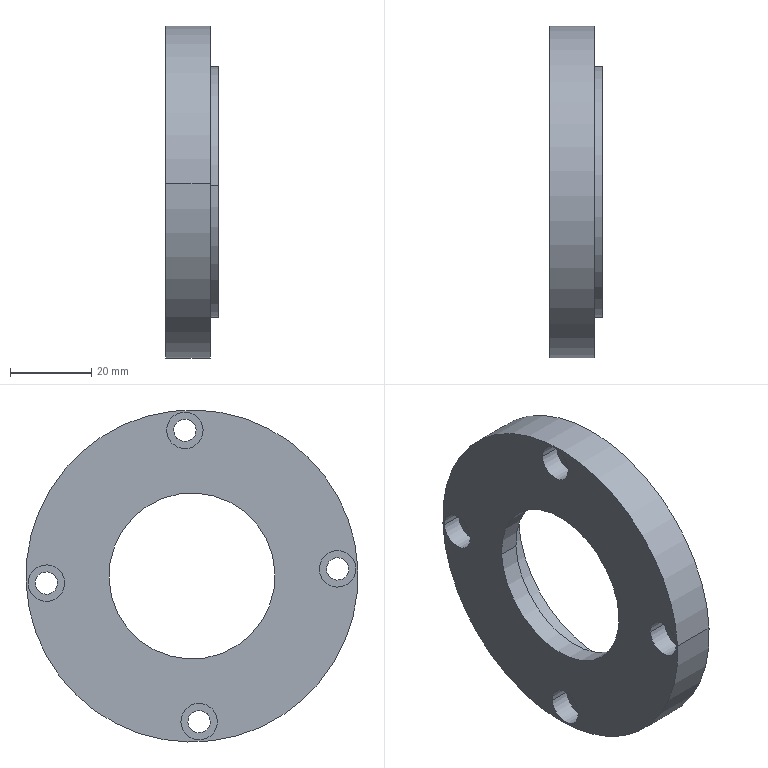Component | SolidWorks | 2-10-10WorkpieceAxisAssembly-1_2-10-3BearingSideCover-2 | 1 solid | 32 faces | box 13 x 82 x 82 mm | volume 36679 mm3 | cylinder 24 | plane 8 | commonest cylinder face diameters 5.5 x8 9 x8 41 x2 55 x2 62 x2 82 x2
STEP:
#1=COLOUR_RGB('',0.7922,0.8196,0.9333);
#2=FILL_AREA_STYLE_COLOUR('',#1);
#3=FILL_AREA_STYLE('',(#2));
#4=SURFACE_STYLE_FILL_AREA(#3);
#5=SURFACE_SIDE_STYLE('',(#4));
#6=SURFACE_STYLE_USAGE(.BOTH.,#5);
#7=PRESENTATION_STYLE_ASSIGNMENT((#6));
#8=CARTESIAN_POINT('',(-18.811,-0.2038,1.421));
#9=VERTEX_POINT('',#8);
#10=CARTESIAN_POINT('',(-18.811,0.01251,1.41));
#11=VERTEX_POINT('',#10);
#12=CARTESIAN_POINT('',(-18.811,-0.09563,1.416));
#13=DIRECTION('',(1.,-0.,0.));
#14=DIRECTION('',(0.,0.9988,-0.04867));
#15=AXIS2_PLACEMENT_3D('',#12,#13,#14);
#16=CIRCLE('',#15,0.1083);
#17=EDGE_CURVE('',#9,#11,#16,.T.);
#18=ORIENTED_EDGE('',*,*,#17,.T.);
#19=CARTESIAN_POINT('',(-19.048,0.01251,1.41));
#20=VERTEX_POINT('',#19);
#21=CARTESIAN_POINT('',(-19.244,0.01251,1.41));
#22=DIRECTION('',(-1.,0.,-0.));
#23=VECTOR('',#22,39.37);
#24=LINE('',#21,#23);
#25=EDGE_CURVE('',#11,#20,#24,.T.);
#26=ORIENTED_EDGE('',*,*,#25,.T.);
#27=CARTESIAN_POINT('',(-19.048,-0.2038,1.421));
#28=VERTEX_POINT('',#27);
#29=CARTESIAN_POINT('',(-19.048,-0.09563,1.416));
#30=DIRECTION('',(-1.,0.,-0.));
#31=DIRECTION('',(0.,-0.9988,0.04867));
#32=AXIS2_PLACEMENT_3D('',#29,#30,#31);
#33=CIRCLE('',#32,0.1083);
#34=EDGE_CURVE('',#20,#28,#33,.T.);
#35=ORIENTED_EDGE('',*,*,#34,.T.);
#36=CARTESIAN_POINT('',(-19.244,-0.2038,1.421));
#37=DIRECTION('',(-1.,0.,-0.));
#38=VECTOR('',#37,39.37);
#39=LINE('',#36,#38);
#40=EDGE_CURVE('',#9,#28,#39,.T.);
#41=ORIENTED_EDGE('',*,*,#40,.F.);
#42=EDGE_LOOP('',(#18,#26,#35,#41));
#43=FACE_OUTER_BOUND('',#42,.T.);
#44=CARTESIAN_POINT('',(-19.244,-0.09563,1.416));
#45=DIRECTION('',(-1.,0.,-0.));
#46=DIRECTION('',(0.,-0.9988,0.04867));
#47=AXIS2_PLACEMENT_3D('',#44,#45,#46);
#48=CYLINDRICAL_SURFACE('',#47,0.1083);
#49=ADVANCED_FACE('',(#43),#48,.F.);
#50=CARTESIAN_POINT('',(-19.048,0.08133,1.407));
#51=VERTEX_POINT('',#50);
#52=CARTESIAN_POINT('',(-19.048,-0.2726,1.424));
#53=VERTEX_POINT('',#52);
#54=CARTESIAN_POINT('',(-19.048,-0.09563,1.416));
#55=DIRECTION('',(-1.,0.,-0.));
#56=DIRECTION('',(0.,-0.9988,0.04867));
#57=AXIS2_PLACEMENT_3D('',#54,#55,#56);
#58=CIRCLE('',#57,0.1772);
#59=EDGE_CURVE('',#51,#53,#58,.T.);
#60=ORIENTED_EDGE('',*,*,#59,.F.);
#61=CARTESIAN_POINT('',(-19.244,0.08133,1.407));
#62=VERTEX_POINT('',#61);
#63=CARTESIAN_POINT('',(-19.244,0.08133,1.407));
#64=DIRECTION('',(-1.,0.,-0.));
#65=VECTOR('',#64,39.37);
#66=LINE('',#63,#65);
#67=EDGE_CURVE('',#51,#62,#66,.T.);
#68=ORIENTED_EDGE('',*,*,#67,.T.);
#69=CARTESIAN_POINT('',(-19.244,-0.2726,1.424));
#70=VERTEX_POINT('',#69);
#71=CARTESIAN_POINT('',(-19.244,-0.09563,1.416));
#72=DIRECTION('',(-1.,0.,-0.));
#73=DIRECTION('',(0.,-0.9988,0.04867));
#74=AXIS2_PLACEMENT_3D('',#71,#72,#73);
#75=CIRCLE('',#74,0.1772);
#76=EDGE_CURVE('',#62,#70,#75,.T.);
#77=ORIENTED_EDGE('',*,*,#76,.T.);
#78=CARTESIAN_POINT('',(-19.244,-0.2726,1.424));
#79=DIRECTION('',(-1.,0.,-0.));
#80=VECTOR('',#79,39.37);
#81=LINE('',#78,#80);
#82=EDGE_CURVE('',#53,#70,#81,.T.);
#83=ORIENTED_EDGE('',*,*,#82,.F.);
#84=EDGE_LOOP('',(#60,#68,#77,#83));
#85=FACE_OUTER_BOUND('',#84,.T.);
#86=CARTESIAN_POINT('',(-19.244,-0.09563,1.416));
#87=DIRECTION('',(-1.,0.,-0.));
#88=DIRECTION('',(0.,-0.9988,0.04867));
#89=AXIS2_PLACEMENT_3D('',#86,#87,#88);
#90=CYLINDRICAL_SURFACE('',#89,0.1772);
#91=ADVANCED_FACE('',(#85),#90,.F.);
#92=CARTESIAN_POINT('',(-18.811,-1.688,0.07425));
#93=VERTEX_POINT('',#92);
#94=CARTESIAN_POINT('',(-18.811,-1.472,0.06371));
#95=VERTEX_POINT('',#94);
#96=CARTESIAN_POINT('',(-18.811,-1.58,0.06898));
#97=DIRECTION('',(1.,-0.,0.));
#98=DIRECTION('',(0.,0.9988,-0.04867));
#99=AXIS2_PLACEMENT_3D('',#96,#97,#98);
#100=CIRCLE('',#99,0.1083);
#101=EDGE_CURVE('',#93,#95,#100,.T.);
#102=ORIENTED_EDGE('',*,*,#101,.T.);
#103=CARTESIAN_POINT('',(-19.048,-1.472,0.06371));
#104=VERTEX_POINT('',#103);
#105=CARTESIAN_POINT('',(-19.244,-1.472,0.06371));
#106=DIRECTION('',(-1.,0.,-0.));
#107=VECTOR('',#106,39.37);
#108=LINE('',#105,#107);
#109=EDGE_CURVE('',#95,#104,#108,.T.);
#110=ORIENTED_EDGE('',*,*,#109,.T.);
#111=CARTESIAN_POINT('',(-19.048,-1.688,0.07425));
#112=VERTEX_POINT('',#111);
#113=CARTESIAN_POINT('',(-19.048,-1.58,0.06898));
#114=DIRECTION('',(-1.,0.,-0.));
#115=DIRECTION('',(0.,-0.9988,0.04867));
#116=AXIS2_PLACEMENT_3D('',#113,#114,#115);
#117=CIRCLE('',#116,0.1083);
#118=EDGE_CURVE('',#104,#112,#117,.T.);
#119=ORIENTED_EDGE('',*,*,#118,.T.);
#120=CARTESIAN_POINT('',(-19.244,-1.688,0.07425));
#121=DIRECTION('',(-1.,0.,-0.));
#122=VECTOR('',#121,39.37);
#123=LINE('',#120,#122);
#124=EDGE_CURVE('',#93,#112,#123,.T.);
#125=ORIENTED_EDGE('',*,*,#124,.F.);
#126=EDGE_LOOP('',(#102,#110,#119,#125));
#127=FACE_OUTER_BOUND('',#126,.T.);
#128=CARTESIAN_POINT('',(-19.244,-1.58,0.06898));
#129=DIRECTION('',(-1.,0.,-0.));
#130=DIRECTION('',(0.,-0.9988,0.04867));
#131=AXIS2_PLACEMENT_3D('',#128,#129,#130);
#132=CYLINDRICAL_SURFACE('',#131,0.1083);
#133=ADVANCED_FACE('',(#127),#132,.F.);
#134=CARTESIAN_POINT('',(-19.048,-1.403,0.06035));
#135=VERTEX_POINT('',#134);
#136=CARTESIAN_POINT('',(-19.048,-1.757,0.0776));
#137=VERTEX_POINT('',#136);
#138=CARTESIAN_POINT('',(-19.048,-1.58,0.06898));
#139=DIRECTION('',(-1.,0.,-0.));
#140=DIRECTION('',(0.,-0.9988,0.04867));
#141=AXIS2_PLACEMENT_3D('',#138,#139,#140);
#142=CIRCLE('',#141,0.1772);
#143=EDGE_CURVE('',#135,#137,#142,.T.);
#144=ORIENTED_EDGE('',*,*,#143,.F.);
#145=CARTESIAN_POINT('',(-19.244,-1.403,0.06035));
#146=VERTEX_POINT('',#145);
#147=CARTESIAN_POINT('',(-19.244,-1.403,0.06035));
#148=DIRECTION('',(-1.,0.,-0.));
#149=VECTOR('',#148,39.37);
#150=LINE('',#147,#149);
#151=EDGE_CURVE('',#135,#146,#150,.T.);
#152=ORIENTED_EDGE('',*,*,#151,.T.);
#153=CARTESIAN_POINT('',(-19.244,-1.757,0.0776));
#154=VERTEX_POINT('',#153);
#155=CARTESIAN_POINT('',(-19.244,-1.58,0.06898));
#156=DIRECTION('',(-1.,0.,-0.));
#157=DIRECTION('',(0.,-0.9988,0.04867));
#158=AXIS2_PLACEMENT_3D('',#155,#156,#157);
#159=CIRCLE('',#158,0.1772);
#160=EDGE_CURVE('',#146,#154,#159,.T.);
#161=ORIENTED_EDGE('',*,*,#160,.T.);
#162=CARTESIAN_POINT('',(-19.244,-1.757,0.0776));
#163=DIRECTION('',(-1.,0.,-0.));
#164=VECTOR('',#163,39.37);
#165=LINE('',#162,#164);
#166=EDGE_CURVE('',#137,#154,#165,.T.);
#167=ORIENTED_EDGE('',*,*,#166,.F.);
#168=EDGE_LOOP('',(#144,#152,#161,#167));
#169=FACE_OUTER_BOUND('',#168,.T.);
#170=CARTESIAN_POINT('',(-19.244,-1.58,0.06898));
#171=DIRECTION('',(-1.,0.,-0.));
#172=DIRECTION('',(0.,-0.9988,0.04867));
#173=AXIS2_PLACEMENT_3D('',#170,#171,#172);
#174=CYLINDRICAL_SURFACE('',#173,0.1772);
#175=ADVANCED_FACE('',(#169),#174,.F.);
#176=CARTESIAN_POINT('',(-18.811,-0.3417,-1.41));
#177=VERTEX_POINT('',#176);
#178=CARTESIAN_POINT('',(-18.811,-0.1254,-1.421));
#179=VERTEX_POINT('',#178);
#180=CARTESIAN_POINT('',(-18.811,-0.2336,-1.416));
#181=DIRECTION('',(1.,-0.,0.));
#182=DIRECTION('',(0.,0.9988,-0.04867));
#183=AXIS2_PLACEMENT_3D('',#180,#181,#182);
#184=CIRCLE('',#183,0.1083);
#185=EDGE_CURVE('',#177,#179,#184,.T.);
#186=ORIENTED_EDGE('',*,*,#185,.T.);
#187=CARTESIAN_POINT('',(-19.048,-0.1254,-1.421));
#188=VERTEX_POINT('',#187);
#189=CARTESIAN_POINT('',(-19.244,-0.1254,-1.421));
#190=DIRECTION('',(-1.,0.,-0.));
#191=VECTOR('',#190,39.37);
#192=LINE('',#189,#191);
#193=EDGE_CURVE('',#179,#188,#192,.T.);
#194=ORIENTED_EDGE('',*,*,#193,.T.);
#195=CARTESIAN_POINT('',(-19.048,-0.3417,-1.41));
#196=VERTEX_POINT('',#195);
#197=CARTESIAN_POINT('',(-19.048,-0.2336,-1.416));
#198=DIRECTION('',(-1.,0.,-0.));
#199=DIRECTION('',(0.,-0.9988,0.04867));
#200=AXIS2_PLACEMENT_3D('',#197,#198,#199);
#201=CIRCLE('',#200,0.1083);
#202=EDGE_CURVE('',#188,#196,#201,.T.);
#203=ORIENTED_EDGE('',*,*,#202,.T.);
#204=CARTESIAN_POINT('',(-19.244,-0.3417,-1.41));
#205=DIRECTION('',(-1.,0.,-0.));
#206=VECTOR('',#205,39.37);
#207=LINE('',#204,#206);
#208=EDGE_CURVE('',#177,#196,#207,.T.);
#209=ORIENTED_EDGE('',*,*,#208,.F.);
#210=EDGE_LOOP('',(#186,#194,#203,#209));
#211=FACE_OUTER_BOUND('',#210,.T.);
#212=CARTESIAN_POINT('',(-19.244,-0.2336,-1.416));
#213=DIRECTION('',(-1.,0.,-0.));
#214=DIRECTION('',(0.,-0.9988,0.04867));
#215=AXIS2_PLACEMENT_3D('',#212,#213,#214);
#216=CYLINDRICAL_SURFACE('',#215,0.1083);
#217=ADVANCED_FACE('',(#211),#216,.F.);
#218=CARTESIAN_POINT('',(-19.048,-0.05663,-1.424));
#219=VERTEX_POINT('',#218);
#220=CARTESIAN_POINT('',(-19.048,-0.4105,-1.407));
#221=VERTEX_POINT('',#220);
#222=CARTESIAN_POINT('',(-19.048,-0.2336,-1.416));
#223=DIRECTION('',(-1.,0.,-0.));
#224=DIRECTION('',(0.,-0.9988,0.04867));
#225=AXIS2_PLACEMENT_3D('',#222,#223,#224);
#226=CIRCLE('',#225,0.1772);
#227=EDGE_CURVE('',#219,#221,#226,.T.);
#228=ORIENTED_EDGE('',*,*,#227,.F.);
#229=CARTESIAN_POINT('',(-19.244,-0.05663,-1.424));
#230=VERTEX_POINT('',#229);
#231=CARTESIAN_POINT('',(-19.244,-0.05663,-1.424));
#232=DIRECTION('',(-1.,0.,-0.));
#233=VECTOR('',#232,39.37);
#234=LINE('',#231,#233);
#235=EDGE_CURVE('',#219,#230,#234,.T.);
#236=ORIENTED_EDGE('',*,*,#235,.T.);
#237=CARTESIAN_POINT('',(-19.244,-0.4105,-1.407));
#238=VERTEX_POINT('',#237);
#239=CARTESIAN_POINT('',(-19.244,-0.2336,-1.416));
#240=DIRECTION('',(-1.,0.,-0.));
#241=DIRECTION('',(0.,-0.9988,0.04867));
#242=AXIS2_PLACEMENT_3D('',#239,#240,#241);
#243=CIRCLE('',#242,0.1772);
#244=EDGE_CURVE('',#230,#238,#243,.T.);
#245=ORIENTED_EDGE('',*,*,#244,.T.);
#246=CARTESIAN_POINT('',(-19.244,-0.4105,-1.407));
#247=DIRECTION('',(-1.,0.,-0.));
#248=VECTOR('',#247,39.37);
#249=LINE('',#246,#248);
#250=EDGE_CURVE('',#221,#238,#249,.T.);
#251=ORIENTED_EDGE('',*,*,#250,.F.);
#252=EDGE_LOOP('',(#228,#236,#245,#251));
#253=FACE_OUTER_BOUND('',#252,.T.);
#254=CARTESIAN_POINT('',(-19.244,-0.2336,-1.416));
#255=DIRECTION('',(-1.,0.,-0.));
#256=DIRECTION('',(0.,-0.9988,0.04867));
#257=AXIS2_PLACEMENT_3D('',#254,#255,#256);
#258=CYLINDRICAL_SURFACE('',#257,0.1772);
#259=ADVANCED_FACE('',(#253),#258,.F.);
#260=CARTESIAN_POINT('',(-18.811,1.143,-0.06371));
#261=VERTEX_POINT('',#260);
#262=CARTESIAN_POINT('',(-18.811,1.359,-0.07425));
#263=VERTEX_POINT('',#262);
#264=CARTESIAN_POINT('',(-18.811,1.251,-0.06898));
#265=DIRECTION('',(1.,-0.,0.));
#266=DIRECTION('',(0.,0.9988,-0.04867));
#267=AXIS2_PLACEMENT_3D('',#264,#265,#266);
#268=CIRCLE('',#267,0.1083);
#269=EDGE_CURVE('',#261,#263,#268,.T.);
#270=ORIENTED_EDGE('',*,*,#269,.T.);
#271=CARTESIAN_POINT('',(-19.048,1.359,-0.07425));
#272=VERTEX_POINT('',#271);
#273=CARTESIAN_POINT('',(-19.244,1.359,-0.07425));
#274=DIRECTION('',(-1.,0.,-0.));
#275=VECTOR('',#274,39.37);
#276=LINE('',#273,#275);
#277=EDGE_CURVE('',#263,#272,#276,.T.);
#278=ORIENTED_EDGE('',*,*,#277,.T.);
#279=CARTESIAN_POINT('',(-19.048,1.143,-0.06371));
#280=VERTEX_POINT('',#279);
#281=CARTESIAN_POINT('',(-19.048,1.251,-0.06898));
#282=DIRECTION('',(-1.,0.,-0.));
#283=DIRECTION('',(0.,-0.9988,0.04867));
#284=AXIS2_PLACEMENT_3D('',#281,#282,#283);
#285=CIRCLE('',#284,0.1083);
#286=EDGE_CURVE('',#272,#280,#285,.T.);
#287=ORIENTED_EDGE('',*,*,#286,.T.);
#288=CARTESIAN_POINT('',(-19.244,1.143,-0.06371));
#289=DIRECTION('',(-1.,0.,-0.));
#290=VECTOR('',#289,39.37);
#291=LINE('',#288,#290);
#292=EDGE_CURVE('',#261,#280,#291,.T.);
#293=ORIENTED_EDGE('',*,*,#292,.F.);
#294=EDGE_LOOP('',(#270,#278,#287,#293));
#295=FACE_OUTER_BOUND('',#294,.T.);
#296=CARTESIAN_POINT('',(-19.244,1.251,-0.06898));
#297=DIRECTION('',(-1.,0.,-0.));
#298=DIRECTION('',(0.,-0.9988,0.04867));
#299=AXIS2_PLACEMENT_3D('',#296,#297,#298);
#300=CYLINDRICAL_SURFACE('',#299,0.1083);
#301=ADVANCED_FACE('',(#295),#300,.F.);
#302=CARTESIAN_POINT('',(-19.048,1.428,-0.0776));
#303=VERTEX_POINT('',#302);
#304=CARTESIAN_POINT('',(-19.048,1.074,-0.06035));
#305=VERTEX_POINT('',#304);
#306=CARTESIAN_POINT('',(-19.048,1.251,-0.06898));
#307=DIRECTION('',(-1.,0.,-0.));
#308=DIRECTION('',(0.,-0.9988,0.04867));
#309=AXIS2_PLACEMENT_3D('',#306,#307,#308);
#310=CIRCLE('',#309,0.1772);
#311=EDGE_CURVE('',#303,#305,#310,.T.);
#312=ORIENTED_EDGE('',*,*,#311,.F.);
#313=CARTESIAN_POINT('',(-19.244,1.428,-0.0776));
#314=VERTEX_POINT('',#313);
#315=CARTESIAN_POINT('',(-19.244,1.428,-0.0776));
#316=DIRECTION('',(-1.,0.,-0.));
#317=VECTOR('',#316,39.37);
#318=LINE('',#315,#317);
#319=EDGE_CURVE('',#303,#314,#318,.T.);
#320=ORIENTED_EDGE('',*,*,#319,.T.);
#321=CARTESIAN_POINT('',(-19.244,1.074,-0.06035));
#322=VERTEX_POINT('',#321);
#323=CARTESIAN_POINT('',(-19.244,1.251,-0.06898));
#324=DIRECTION('',(-1.,0.,-0.));
#325=DIRECTION('',(0.,-0.9988,0.04867));
#326=AXIS2_PLACEMENT_3D('',#323,#324,#325);
#327=CIRCLE('',#326,0.1772);
#328=EDGE_CURVE('',#314,#322,#327,.T.);
#329=ORIENTED_EDGE('',*,*,#328,.T.);
#330=CARTESIAN_POINT('',(-19.244,1.074,-0.06035));
#331=DIRECTION('',(-1.,0.,-0.));
#332=VECTOR('',#331,39.37);
#333=LINE('',#330,#332);
#334=EDGE_CURVE('',#305,#322,#333,.T.);
#335=ORIENTED_EDGE('',*,*,#334,.F.);
#336=EDGE_LOOP('',(#312,#320,#329,#335));
#337=FACE_OUTER_BOUND('',#336,.T.);
#338=CARTESIAN_POINT('',(-19.244,1.251,-0.06898));
#339=DIRECTION('',(-1.,0.,-0.));
#340=DIRECTION('',(0.,-0.9988,0.04867));
#341=AXIS2_PLACEMENT_3D('',#338,#339,#340);
#342=CYLINDRICAL_SURFACE('',#341,0.1772);
#343=ADVANCED_FACE('',(#337),#342,.F.);
#344=CARTESIAN_POINT('',(-19.244,-0.9707,0.03928));
#345=VERTEX_POINT('',#344);
#346=CARTESIAN_POINT('',(-19.244,0.6415,-0.03928));
#347=VERTEX_POINT('',#346);
#348=CARTESIAN_POINT('',(-19.244,-0.1646,-0.));
#349=DIRECTION('',(1.,-0.,0.));
#350=DIRECTION('',(0.,0.9988,-0.04867));
#351=AXIS2_PLACEMENT_3D('',#348,#349,#350);
#352=CIRCLE('',#351,0.8071);
#353=EDGE_CURVE('',#345,#347,#352,.T.);
#354=ORIENTED_EDGE('',*,*,#353,.F.);
#355=CARTESIAN_POINT('',(-19.048,-0.9707,0.03928));
#356=VERTEX_POINT('',#355);
#357=CARTESIAN_POINT('',(-18.258,-0.9707,0.03928));
#358=DIRECTION('',(1.,-0.,0.));
#359=VECTOR('',#358,39.37);
#360=LINE('',#357,#359);
#361=EDGE_CURVE('',#345,#356,#360,.T.);
#362=ORIENTED_EDGE('',*,*,#361,.T.);
#363=CARTESIAN_POINT('',(-19.048,0.6415,-0.03928));
#364=VERTEX_POINT('',#363);
#365=CARTESIAN_POINT('',(-19.048,-0.1646,-0.));
#366=DIRECTION('',(1.,-0.,0.));
#367=DIRECTION('',(0.,0.9988,-0.04867));
#368=AXIS2_PLACEMENT_3D('',#365,#366,#367);
#369=CIRCLE('',#368,0.8071);
#370=EDGE_CURVE('',#356,#364,#369,.T.);
#371=ORIENTED_EDGE('',*,*,#370,.T.);
#372=CARTESIAN_POINT('',(-18.258,0.6415,-0.03928));
#373=DIRECTION('',(1.,-0.,0.));
#374=VECTOR('',#373,39.37);
#375=LINE('',#372,#374);
#376=EDGE_CURVE('',#347,#364,#375,.T.);
#377=ORIENTED_EDGE('',*,*,#376,.F.);
#378=EDGE_LOOP('',(#354,#362,#371,#377));
#379=FACE_OUTER_BOUND('',#378,.T.);
#380=CARTESIAN_POINT('',(-18.258,-0.1646,-0.));
#381=DIRECTION('',(1.,-0.,0.));
#382=DIRECTION('',(0.,0.9988,-0.04867));
#383=AXIS2_PLACEMENT_3D('',#380,#381,#382);
#384=CYLINDRICAL_SURFACE('',#383,0.8071);
#385=ADVANCED_FACE('',(#379),#384,.F.);
#386=CARTESIAN_POINT('',(-19.048,-1.246,0.05269));
#387=VERTEX_POINT('',#386);
#388=CARTESIAN_POINT('',(-19.048,0.9168,-0.05269));
#389=VERTEX_POINT('',#388);
#390=CARTESIAN_POINT('',(-19.048,-0.1646,-0.));
#391=DIRECTION('',(1.,-0.,0.));
#392=DIRECTION('',(0.,0.9988,-0.04867));
#393=AXIS2_PLACEMENT_3D('',#390,#391,#392);
#394=CIRCLE('',#393,1.083);
#395=EDGE_CURVE('',#387,#389,#394,.T.);
#396=ORIENTED_EDGE('',*,*,#395,.F.);
#397=CARTESIAN_POINT('',(-18.733,-1.246,0.05269));
#398=VERTEX_POINT('',#397);
#399=CARTESIAN_POINT('',(-18.258,-1.246,0.05269));
#400=DIRECTION('',(1.,-0.,0.));
#401=VECTOR('',#400,39.37);
#402=LINE('',#399,#401);
#403=EDGE_CURVE('',#387,#398,#402,.T.);
#404=ORIENTED_EDGE('',*,*,#403,.T.);
#405=CARTESIAN_POINT('',(-18.733,0.9168,-0.05269));
#406=VERTEX_POINT('',#405);
#407=CARTESIAN_POINT('',(-18.733,-0.1646,-0.));
#408=DIRECTION('',(1.,-0.,0.));
#409=DIRECTION('',(0.,0.9988,-0.04867));
#410=AXIS2_PLACEMENT_3D('',#407,#408,#409);
#411=CIRCLE('',#410,1.083);
#412=EDGE_CURVE('',#398,#406,#411,.T.);
#413=ORIENTED_EDGE('',*,*,#412,.T.);
#414=CARTESIAN_POINT('',(-18.258,0.9168,-0.05269));
#415=DIRECTION('',(1.,-0.,0.));
#416=VECTOR('',#415,39.37);
#417=LINE('',#414,#416);
#418=EDGE_CURVE('',#389,#406,#417,.T.);
#419=ORIENTED_EDGE('',*,*,#418,.F.);
#420=EDGE_LOOP('',(#396,#404,#413,#419));
#421=FACE_OUTER_BOUND('',#420,.T.);
#422=CARTESIAN_POINT('',(-18.258,-0.1646,-0.));
#423=DIRECTION('',(1.,-0.,0.));
#424=DIRECTION('',(0.,0.9988,-0.04867));
#425=AXIS2_PLACEMENT_3D('',#422,#423,#424);
#426=CYLINDRICAL_SURFACE('',#425,1.083);
#427=ADVANCED_FACE('',(#421),#426,.F.);
#428=CARTESIAN_POINT('',(-18.811,1.054,-0.0594));
#429=VERTEX_POINT('',#428);
#430=CARTESIAN_POINT('',(-18.811,-1.384,0.0594));
#431=VERTEX_POINT('',#430);
#432=CARTESIAN_POINT('',(-18.811,-0.1646,-0.));
#433=DIRECTION('',(1.,-0.,0.));
#434=DIRECTION('',(0.,0.9988,-0.04867));
#435=AXIS2_PLACEMENT_3D('',#432,#433,#434);
#436=CIRCLE('',#435,1.22);
#437=EDGE_CURVE('',#429,#431,#436,.T.);
#438=ORIENTED_EDGE('',*,*,#437,.T.);
#439=CARTESIAN_POINT('',(-18.733,-1.384,0.0594));
#440=VERTEX_POINT('',#439);
#441=CARTESIAN_POINT('',(-18.258,-1.384,0.0594));
#442=DIRECTION('',(1.,-0.,0.));
#443=VECTOR('',#442,39.37);
#444=LINE('',#441,#443);
#445=EDGE_CURVE('',#431,#440,#444,.T.);
#446=ORIENTED_EDGE('',*,*,#445,.T.);
#447=CARTESIAN_POINT('',(-18.733,1.054,-0.0594));
#448=VERTEX_POINT('',#447);
#449=CARTESIAN_POINT('',(-18.733,-0.1646,-0.));
#450=DIRECTION('',(1.,-0.,0.));
#451=DIRECTION('',(0.,0.9988,-0.04867));
#452=AXIS2_PLACEMENT_3D('',#449,#450,#451);
#453=CIRCLE('',#452,1.22);
#454=EDGE_CURVE('',#448,#440,#453,.T.);
#455=ORIENTED_EDGE('',*,*,#454,.F.);
#456=CARTESIAN_POINT('',(-18.258,1.054,-0.0594));
#457=DIRECTION('',(1.,-0.,0.));
#458=VECTOR('',#457,39.37);
#459=LINE('',#456,#458);
#460=EDGE_CURVE('',#429,#448,#459,.T.);
#461=ORIENTED_EDGE('',*,*,#460,.F.);
#462=EDGE_LOOP('',(#438,#446,#455,#461));
#463=FACE_OUTER_BOUND('',#462,.T.);
#464=CARTESIAN_POINT('',(-18.258,-0.1646,-0.));
#465=DIRECTION('',(1.,-0.,0.));
#466=DIRECTION('',(0.,0.9988,-0.04867));
#467=AXIS2_PLACEMENT_3D('',#464,#465,#466);
#468=CYLINDRICAL_SURFACE('',#467,1.22);
#469=ADVANCED_FACE('',(#463),#468,.T.);
#470=CARTESIAN_POINT('',(-19.244,1.448,-0.07856));
#471=VERTEX_POINT('',#470);
#472=CARTESIAN_POINT('',(-19.244,-1.777,0.07856));
#473=VERTEX_POINT('',#472);
#474=CARTESIAN_POINT('',(-19.244,-0.1646,-0.));
#475=DIRECTION('',(1.,-0.,0.));
#476=DIRECTION('',(0.,0.9988,-0.04867));
#477=AXIS2_PLACEMENT_3D('',#474,#475,#476);
#478=CIRCLE('',#477,1.614);
#479=EDGE_CURVE('',#471,#473,#478,.T.);
#480=ORIENTED_EDGE('',*,*,#479,.T.);
#481=CARTESIAN_POINT('',(-18.811,-1.777,0.07856));
#482=VERTEX_POINT('',#481);
#483=CARTESIAN_POINT('',(-18.258,-1.777,0.07856));
#484=DIRECTION('',(1.,-0.,0.));
#485=VECTOR('',#484,39.37);
#486=LINE('',#483,#485);
#487=EDGE_CURVE('',#473,#482,#486,.T.);
#488=ORIENTED_EDGE('',*,*,#487,.T.);
#489=CARTESIAN_POINT('',(-18.811,1.448,-0.07856));
#490=VERTEX_POINT('',#489);
#491=CARTESIAN_POINT('',(-18.811,-0.1646,-0.));
#492=DIRECTION('',(1.,-0.,0.));
#493=DIRECTION('',(0.,0.9988,-0.04867));
#494=AXIS2_PLACEMENT_3D('',#491,#492,#493);
#495=CIRCLE('',#494,1.614);
#496=EDGE_CURVE('',#490,#482,#495,.T.);
#497=ORIENTED_EDGE('',*,*,#496,.F.);
#498=CARTESIAN_POINT('',(-18.258,1.448,-0.07856));
#499=DIRECTION('',(1.,-0.,0.));
#500=VECTOR('',#499,39.37);
#501=LINE('',#498,#500);
#502=EDGE_CURVE('',#471,#490,#501,.T.);
#503=ORIENTED_EDGE('',*,*,#502,.F.);
#504=EDGE_LOOP('',(#480,#488,#497,#503));
#505=FACE_OUTER_BOUND('',#504,.T.);
#506=CARTESIAN_POINT('',(-18.258,-0.1646,-0.));
#507=DIRECTION('',(1.,-0.,0.));
#508=DIRECTION('',(0.,0.9988,-0.04867));
#509=AXIS2_PLACEMENT_3D('',#506,#507,#508);
#510=CYLINDRICAL_SURFACE('',#509,1.614);
#511=ADVANCED_FACE('',(#505),#510,.T.);
#512=ORIENTED_EDGE('',*,*,#487,.F.);
#513=CARTESIAN_POINT('',(-19.244,-0.1646,-0.));
#514=DIRECTION('',(1.,-0.,0.));
#515=DIRECTION('',(0.,0.9988,-0.04867));
#516=AXIS2_PLACEMENT_3D('',#513,#514,#515);
#517=CIRCLE('',#516,1.614);
#518=EDGE_CURVE('',#473,#471,#517,.T.);
#519=ORIENTED_EDGE('',*,*,#518,.T.);
#520=ORIENTED_EDGE('',*,*,#502,.T.);
#521=CARTESIAN_POINT('',(-18.811,-0.1646,-0.));
#522=DIRECTION('',(1.,-0.,0.));
#523=DIRECTION('',(0.,0.9988,-0.04867));
#524=AXIS2_PLACEMENT_3D('',#521,#522,#523);
#525=CIRCLE('',#524,1.614);
#526=EDGE_CURVE('',#482,#490,#525,.T.);
#527=ORIENTED_EDGE('',*,*,#526,.F.);
#528=EDGE_LOOP('',(#512,#519,#520,#527));
#529=FACE_OUTER_BOUND('',#528,.T.);
#530=CARTESIAN_POINT('',(-18.258,-0.1646,-0.));
#531=DIRECTION('',(1.,-0.,0.));
#532=DIRECTION('',(0.,0.9988,-0.04867));
#533=AXIS2_PLACEMENT_3D('',#530,#531,#532);
#534=CYLINDRICAL_SURFACE('',#533,1.614);
#535=ADVANCED_FACE('',(#529),#534,.T.);
#536=ORIENTED_EDGE('',*,*,#17,.F.);
#537=CARTESIAN_POINT('',(-18.811,-0.09563,1.416));
#538=DIRECTION('',(1.,-0.,0.));
#539=DIRECTION('',(0.,0.9988,-0.04867));
#540=AXIS2_PLACEMENT_3D('',#537,#538,#539);
#541=CIRCLE('',#540,0.1083);
#542=EDGE_CURVE('',#11,#9,#541,.T.);
#543=ORIENTED_EDGE('',*,*,#542,.F.);
#544=EDGE_LOOP('',(#536,#543));
#545=FACE_BOUND('',#544,.T.);
#546=ORIENTED_EDGE('',*,*,#101,.F.);
#547=CARTESIAN_POINT('',(-18.811,-1.58,0.06898));
#548=DIRECTION('',(1.,-0.,0.));
#549=DIRECTION('',(0.,0.9988,-0.04867));
#550=AXIS2_PLACEMENT_3D('',#547,#548,#549);
#551=CIRCLE('',#550,0.1083);
#552=EDGE_CURVE('',#95,#93,#551,.T.);
#553=ORIENTED_EDGE('',*,*,#552,.F.);
#554=EDGE_LOOP('',(#546,#553));
#555=FACE_BOUND('',#554,.T.);
#556=ORIENTED_EDGE('',*,*,#185,.F.);
#557=CARTESIAN_POINT('',(-18.811,-0.2336,-1.416));
#558=DIRECTION('',(1.,-0.,0.));
#559=DIRECTION('',(0.,0.9988,-0.04867));
#560=AXIS2_PLACEMENT_3D('',#557,#558,#559);
#561=CIRCLE('',#560,0.1083);
#562=EDGE_CURVE('',#179,#177,#561,.T.);
#563=ORIENTED_EDGE('',*,*,#562,.F.);
#564=EDGE_LOOP('',(#556,#563));
#565=FACE_BOUND('',#564,.T.);
#566=ORIENTED_EDGE('',*,*,#269,.F.);
#567=CARTESIAN_POINT('',(-18.811,1.251,-0.06898));
#568=DIRECTION('',(1.,-0.,0.));
#569=DIRECTION('',(0.,0.9988,-0.04867));
#570=AXIS2_PLACEMENT_3D('',#567,#568,#569);
#571=CIRCLE('',#570,0.1083);
#572=EDGE_CURVE('',#263,#261,#571,.T.);
#573=ORIENTED_EDGE('',*,*,#572,.F.);
#574=EDGE_LOOP('',(#566,#573));
#575=FACE_BOUND('',#574,.T.);
#576=ORIENTED_EDGE('',*,*,#496,.T.);
#577=ORIENTED_EDGE('',*,*,#526,.T.);
#578=EDGE_LOOP('',(#576,#577));
#579=FACE_OUTER_BOUND('',#578,.T.);
#580=ORIENTED_EDGE('',*,*,#437,.F.);
#581=CARTESIAN_POINT('',(-18.811,-0.1646,-0.));
#582=DIRECTION('',(1.,-0.,0.));
#583=DIRECTION('',(0.,0.9988,-0.04867));
#584=AXIS2_PLACEMENT_3D('',#581,#582,#583);
#585=CIRCLE('',#584,1.22);
#586=EDGE_CURVE('',#431,#429,#585,.T.);
#587=ORIENTED_EDGE('',*,*,#586,.F.);
#588=EDGE_LOOP('',(#580,#587));
#589=FACE_BOUND('',#588,.T.);
#590=CARTESIAN_POINT('',(-18.811,1.448,-0.07856));
#591=DIRECTION('',(1.,-0.,0.));
#592=DIRECTION('',(0.,0.9988,-0.04867));
#593=AXIS2_PLACEMENT_3D('',#590,#591,#592);
#594=PLANE('',#593);
#595=ADVANCED_FACE('',(#545,#555,#565,#575,#579,#589),#594,.T.);
#596=ORIENTED_EDGE('',*,*,#445,.F.);
#597=ORIENTED_EDGE('',*,*,#586,.T.);
#598=ORIENTED_EDGE('',*,*,#460,.T.);
#599=CARTESIAN_POINT('',(-18.733,-0.1646,-0.));
#600=DIRECTION('',(1.,-0.,0.));
#601=DIRECTION('',(0.,0.9988,-0.04867));
#602=AXIS2_PLACEMENT_3D('',#599,#600,#601);
#603=CIRCLE('',#602,1.22);
#604=EDGE_CURVE('',#440,#448,#603,.T.);
#605=ORIENTED_EDGE('',*,*,#604,.F.);
#606=EDGE_LOOP('',(#596,#597,#598,#605));
#607=FACE_OUTER_BOUND('',#606,.T.);
#608=CARTESIAN_POINT('',(-18.258,-0.1646,-0.));
#609=DIRECTION('',(1.,-0.,0.));
#610=DIRECTION('',(0.,0.9988,-0.04867));
#611=AXIS2_PLACEMENT_3D('',#608,#609,#610);
#612=CYLINDRICAL_SURFACE('',#611,1.22);
#613=ADVANCED_FACE('',(#607),#612,.T.);
#614=ORIENTED_EDGE('',*,*,#454,.T.);
#615=ORIENTED_EDGE('',*,*,#604,.T.);
#616=EDGE_LOOP('',(#614,#615));
#617=FACE_OUTER_BOUND('',#616,.T.);
#618=CARTESIAN_POINT('',(-18.733,-0.1646,-0.));
#619=DIRECTION('',(1.,-0.,0.));
#620=DIRECTION('',(0.,0.9988,-0.04867));
#621=AXIS2_PLACEMENT_3D('',#618,#619,#620);
#622=CIRCLE('',#621,1.083);
#623=EDGE_CURVE('',#406,#398,#622,.T.);
#624=ORIENTED_EDGE('',*,*,#623,.F.);
#625=ORIENTED_EDGE('',*,*,#412,.F.);
#626=EDGE_LOOP('',(#624,#625));
#627=FACE_BOUND('',#626,.T.);
#628=CARTESIAN_POINT('',(-18.733,1.054,-0.0594));
#629=DIRECTION('',(1.,-0.,0.));
#630=DIRECTION('',(0.,0.9988,-0.04867));
#631=AXIS2_PLACEMENT_3D('',#628,#629,#630);
#632=PLANE('',#631);
#633=ADVANCED_FACE('',(#617,#627),#632,.T.);
#634=ORIENTED_EDGE('',*,*,#403,.F.);
#635=CARTESIAN_POINT('',(-19.048,-0.1646,-0.));
#636=DIRECTION('',(1.,-0.,0.));
#637=DIRECTION('',(0.,0.9988,-0.04867));
#638=AXIS2_PLACEMENT_3D('',#635,#636,#637);
#639=CIRCLE('',#638,1.083);
#640=EDGE_CURVE('',#389,#387,#639,.T.);
#641=ORIENTED_EDGE('',*,*,#640,.F.);
#642=ORIENTED_EDGE('',*,*,#418,.T.);
#643=ORIENTED_EDGE('',*,*,#623,.T.);
#644=EDGE_LOOP('',(#634,#641,#642,#643));
#645=FACE_OUTER_BOUND('',#644,.T.);
#646=CARTESIAN_POINT('',(-18.258,-0.1646,-0.));
#647=DIRECTION('',(1.,-0.,0.));
#648=DIRECTION('',(0.,0.9988,-0.04867));
#649=AXIS2_PLACEMENT_3D('',#646,#647,#648);
#650=CYLINDRICAL_SURFACE('',#649,1.083);
#651=ADVANCED_FACE('',(#645),#650,.F.);
#652=ORIENTED_EDGE('',*,*,#640,.T.);
#653=ORIENTED_EDGE('',*,*,#395,.T.);
#654=EDGE_LOOP('',(#652,#653));
#655=FACE_OUTER_BOUND('',#654,.T.);
#656=CARTESIAN_POINT('',(-19.048,-0.1646,-0.));
#657=DIRECTION('',(1.,-0.,0.));
#658=DIRECTION('',(0.,0.9988,-0.04867));
#659=AXIS2_PLACEMENT_3D('',#656,#657,#658);
#660=CIRCLE('',#659,0.8071);
#661=EDGE_CURVE('',#364,#356,#660,.T.);
#662=ORIENTED_EDGE('',*,*,#661,.F.);
#663=ORIENTED_EDGE('',*,*,#370,.F.);
#664=EDGE_LOOP('',(#662,#663));
#665=FACE_BOUND('',#664,.T.);
#666=CARTESIAN_POINT('',(-19.048,0.9168,-0.05269));
#667=DIRECTION('',(1.,-0.,0.));
#668=DIRECTION('',(0.,0.9988,-0.04867));
#669=AXIS2_PLACEMENT_3D('',#666,#667,#668);
#670=PLANE('',#669);
#671=ADVANCED_FACE('',(#655,#665),#670,.T.);
#672=ORIENTED_EDGE('',*,*,#361,.F.);
#673=CARTESIAN_POINT('',(-19.244,-0.1646,-0.));
#674=DIRECTION('',(1.,-0.,0.));
#675=DIRECTION('',(0.,0.9988,-0.04867));
#676=AXIS2_PLACEMENT_3D('',#673,#674,#675);
#677=CIRCLE('',#676,0.8071);
#678=EDGE_CURVE('',#347,#345,#677,.T.);
#679=ORIENTED_EDGE('',*,*,#678,.F.);
#680=ORIENTED_EDGE('',*,*,#376,.T.);
#681=ORIENTED_EDGE('',*,*,#661,.T.);
#682=EDGE_LOOP('',(#672,#679,#680,#681));
#683=FACE_OUTER_BOUND('',#682,.T.);
#684=CARTESIAN_POINT('',(-18.258,-0.1646,-0.));
#685=DIRECTION('',(1.,-0.,0.));
#686=DIRECTION('',(0.,0.9988,-0.04867));
#687=AXIS2_PLACEMENT_3D('',#684,#685,#686);
#688=CYLINDRICAL_SURFACE('',#687,0.8071);
#689=ADVANCED_FACE('',(#683),#688,.F.);
#690=CARTESIAN_POINT('',(-19.244,-0.09563,1.416));
#691=DIRECTION('',(-1.,0.,-0.));
#692=DIRECTION('',(0.,-0.9988,0.04867));
#693=AXIS2_PLACEMENT_3D('',#690,#691,#692);
#694=CIRCLE('',#693,0.1772);
#695=EDGE_CURVE('',#70,#62,#694,.T.);
#696=ORIENTED_EDGE('',*,*,#695,.F.);
#697=ORIENTED_EDGE('',*,*,#76,.F.);
#698=EDGE_LOOP('',(#696,#697));
#699=FACE_BOUND('',#698,.T.);
#700=CARTESIAN_POINT('',(-19.244,-1.58,0.06898));
#701=DIRECTION('',(-1.,0.,-0.));
#702=DIRECTION('',(0.,-0.9988,0.04867));
#703=AXIS2_PLACEMENT_3D('',#700,#701,#702);
#704=CIRCLE('',#703,0.1772);
#705=EDGE_CURVE('',#154,#146,#704,.T.);
#706=ORIENTED_EDGE('',*,*,#705,.F.);
#707=ORIENTED_EDGE('',*,*,#160,.F.);
#708=EDGE_LOOP('',(#706,#707));
#709=FACE_BOUND('',#708,.T.);
#710=CARTESIAN_POINT('',(-19.244,-0.2336,-1.416));
#711=DIRECTION('',(-1.,0.,-0.));
#712=DIRECTION('',(0.,-0.9988,0.04867));
#713=AXIS2_PLACEMENT_3D('',#710,#711,#712);
#714=CIRCLE('',#713,0.1772);
#715=EDGE_CURVE('',#238,#230,#714,.T.);
#716=ORIENTED_EDGE('',*,*,#715,.F.);
#717=ORIENTED_EDGE('',*,*,#244,.F.);
#718=EDGE_LOOP('',(#716,#717));
#719=FACE_BOUND('',#718,.T.);
#720=CARTESIAN_POINT('',(-19.244,1.251,-0.06898));
#721=DIRECTION('',(-1.,0.,-0.));
#722=DIRECTION('',(0.,-0.9988,0.04867));
#723=AXIS2_PLACEMENT_3D('',#720,#721,#722);
#724=CIRCLE('',#723,0.1772);
#725=EDGE_CURVE('',#322,#314,#724,.T.);
#726=ORIENTED_EDGE('',*,*,#725,.F.);
#727=ORIENTED_EDGE('',*,*,#328,.F.);
#728=EDGE_LOOP('',(#726,#727));
#729=FACE_BOUND('',#728,.T.);
#730=ORIENTED_EDGE('',*,*,#678,.T.);
#731=ORIENTED_EDGE('',*,*,#353,.T.);
#732=EDGE_LOOP('',(#730,#731));
#733=FACE_BOUND('',#732,.T.);
#734=ORIENTED_EDGE('',*,*,#479,.F.);
#735=ORIENTED_EDGE('',*,*,#518,.F.);
#736=EDGE_LOOP('',(#734,#735));
#737=FACE_OUTER_BOUND('',#736,.T.);
#738=CARTESIAN_POINT('',(-19.244,0.6415,-0.03928));
#739=DIRECTION('',(-1.,0.,-0.));
#740=DIRECTION('',(-0.,-0.9988,0.04867));
#741=AXIS2_PLACEMENT_3D('',#738,#739,#740);
#742=PLANE('',#741);
#743=ADVANCED_FACE('',(#699,#709,#719,#729,#733,#737),#742,.T.);
#744=ORIENTED_EDGE('',*,*,#319,.F.);
#745=CARTESIAN_POINT('',(-19.048,1.251,-0.06898));
#746=DIRECTION('',(-1.,0.,-0.));
#747=DIRECTION('',(0.,-0.9988,0.04867));
#748=AXIS2_PLACEMENT_3D('',#745,#746,#747);
#749=CIRCLE('',#748,0.1772);
#750=EDGE_CURVE('',#305,#303,#749,.T.);
#751=ORIENTED_EDGE('',*,*,#750,.F.);
#752=ORIENTED_EDGE('',*,*,#334,.T.);
#753=ORIENTED_EDGE('',*,*,#725,.T.);
#754=EDGE_LOOP('',(#744,#751,#752,#753));
#755=FACE_OUTER_BOUND('',#754,.T.);
#756=CARTESIAN_POINT('',(-19.244,1.251,-0.06898));
#757=DIRECTION('',(-1.,0.,-0.));
#758=DIRECTION('',(0.,-0.9988,0.04867));
#759=AXIS2_PLACEMENT_3D('',#756,#757,#758);
#760=CYLINDRICAL_SURFACE('',#759,0.1772);
#761=ADVANCED_FACE('',(#755),#760,.F.);
#762=CARTESIAN_POINT('',(-19.048,1.251,-0.06898));
#763=DIRECTION('',(-1.,0.,-0.));
#764=DIRECTION('',(0.,-0.9988,0.04867));
#765=AXIS2_PLACEMENT_3D('',#762,#763,#764);
#766=CIRCLE('',#765,0.1083);
#767=EDGE_CURVE('',#280,#272,#766,.T.);
#768=ORIENTED_EDGE('',*,*,#767,.F.);
#769=ORIENTED_EDGE('',*,*,#286,.F.);
#770=EDGE_LOOP('',(#768,#769));
#771=FACE_BOUND('',#770,.T.);
#772=ORIENTED_EDGE('',*,*,#750,.T.);
#773=ORIENTED_EDGE('',*,*,#311,.T.);
#774=EDGE_LOOP('',(#772,#773));
#775=FACE_OUTER_BOUND('',#774,.T.);
#776=CARTESIAN_POINT('',(-19.048,1.256,0.03916));
#777=DIRECTION('',(1.,-0.,0.));
#778=DIRECTION('',(0.,0.9988,-0.04867));
#779=AXIS2_PLACEMENT_3D('',#776,#777,#778);
#780=PLANE('',#779);
#781=ADVANCED_FACE('',(#771,#775),#780,.F.);
#782=ORIENTED_EDGE('',*,*,#277,.F.);
#783=ORIENTED_EDGE('',*,*,#572,.T.);
#784=ORIENTED_EDGE('',*,*,#292,.T.);
#785=ORIENTED_EDGE('',*,*,#767,.T.);
#786=EDGE_LOOP('',(#782,#783,#784,#785));
#787=FACE_OUTER_BOUND('',#786,.T.);
#788=CARTESIAN_POINT('',(-19.244,1.251,-0.06898));
#789=DIRECTION('',(-1.,0.,-0.));
#790=DIRECTION('',(0.,-0.9988,0.04867));
#791=AXIS2_PLACEMENT_3D('',#788,#789,#790);
#792=CYLINDRICAL_SURFACE('',#791,0.1083);
#793=ADVANCED_FACE('',(#787),#792,.F.);
#794=ORIENTED_EDGE('',*,*,#235,.F.);
#795=CARTESIAN_POINT('',(-19.048,-0.2336,-1.416));
#796=DIRECTION('',(-1.,0.,-0.));
#797=DIRECTION('',(0.,-0.9988,0.04867));
#798=AXIS2_PLACEMENT_3D('',#795,#796,#797);
#799=CIRCLE('',#798,0.1772);
#800=EDGE_CURVE('',#221,#219,#799,.T.);
#801=ORIENTED_EDGE('',*,*,#800,.F.);
#802=ORIENTED_EDGE('',*,*,#250,.T.);
#803=ORIENTED_EDGE('',*,*,#715,.T.);
#804=EDGE_LOOP('',(#794,#801,#802,#803));
#805=FACE_OUTER_BOUND('',#804,.T.);
#806=CARTESIAN_POINT('',(-19.244,-0.2336,-1.416));
#807=DIRECTION('',(-1.,0.,-0.));
#808=DIRECTION('',(0.,-0.9988,0.04867));
#809=AXIS2_PLACEMENT_3D('',#806,#807,#808);
#810=CYLINDRICAL_SURFACE('',#809,0.1772);
#811=ADVANCED_FACE('',(#805),#810,.F.);
#812=CARTESIAN_POINT('',(-19.048,-0.2336,-1.416));
#813=DIRECTION('',(-1.,0.,-0.));
#814=DIRECTION('',(0.,-0.9988,0.04867));
#815=AXIS2_PLACEMENT_3D('',#812,#813,#814);
#816=CIRCLE('',#815,0.1083);
#817=EDGE_CURVE('',#196,#188,#816,.T.);
#818=ORIENTED_EDGE('',*,*,#817,.F.);
#819=ORIENTED_EDGE('',*,*,#202,.F.);
#820=EDGE_LOOP('',(#818,#819));
#821=FACE_BOUND('',#820,.T.);
#822=ORIENTED_EDGE('',*,*,#800,.T.);
#823=ORIENTED_EDGE('',*,*,#227,.T.);
#824=EDGE_LOOP('',(#822,#823));
#825=FACE_OUTER_BOUND('',#824,.T.);
#826=CARTESIAN_POINT('',(-19.048,-0.2283,-1.308));
#827=DIRECTION('',(1.,-0.,0.));
#828=DIRECTION('',(0.,0.9988,-0.04867));
#829=AXIS2_PLACEMENT_3D('',#826,#827,#828);
#830=PLANE('',#829);
#831=ADVANCED_FACE('',(#821,#825),#830,.F.);
#832=ORIENTED_EDGE('',*,*,#193,.F.);
#833=ORIENTED_EDGE('',*,*,#562,.T.);
#834=ORIENTED_EDGE('',*,*,#208,.T.);
#835=ORIENTED_EDGE('',*,*,#817,.T.);
#836=EDGE_LOOP('',(#832,#833,#834,#835));
#837=FACE_OUTER_BOUND('',#836,.T.);
#838=CARTESIAN_POINT('',(-19.244,-0.2336,-1.416));
#839=DIRECTION('',(-1.,0.,-0.));
#840=DIRECTION('',(0.,-0.9988,0.04867));
#841=AXIS2_PLACEMENT_3D('',#838,#839,#840);
#842=CYLINDRICAL_SURFACE('',#841,0.1083);
#843=ADVANCED_FACE('',(#837),#842,.F.);
#844=ORIENTED_EDGE('',*,*,#151,.F.);
#845=CARTESIAN_POINT('',(-19.048,-1.58,0.06898));
#846=DIRECTION('',(-1.,0.,-0.));
#847=DIRECTION('',(0.,-0.9988,0.04867));
#848=AXIS2_PLACEMENT_3D('',#845,#846,#847);
#849=CIRCLE('',#848,0.1772);
#850=EDGE_CURVE('',#137,#135,#849,.T.);
#851=ORIENTED_EDGE('',*,*,#850,.F.);
#852=ORIENTED_EDGE('',*,*,#166,.T.);
#853=ORIENTED_EDGE('',*,*,#705,.T.);
#854=EDGE_LOOP('',(#844,#851,#852,#853));
#855=FACE_OUTER_BOUND('',#854,.T.);
#856=CARTESIAN_POINT('',(-19.244,-1.58,0.06898));
#857=DIRECTION('',(-1.,0.,-0.));
#858=DIRECTION('',(0.,-0.9988,0.04867));
#859=AXIS2_PLACEMENT_3D('',#856,#857,#858);
#860=CYLINDRICAL_SURFACE('',#859,0.1772);
#861=ADVANCED_FACE('',(#855),#860,.F.);
#862=CARTESIAN_POINT('',(-19.048,-1.58,0.06898));
#863=DIRECTION('',(-1.,0.,-0.));
#864=DIRECTION('',(0.,-0.9988,0.04867));
#865=AXIS2_PLACEMENT_3D('',#862,#863,#864);
#866=CIRCLE('',#865,0.1083);
#867=EDGE_CURVE('',#112,#104,#866,.T.);
#868=ORIENTED_EDGE('',*,*,#867,.F.);
#869=ORIENTED_EDGE('',*,*,#118,.F.);
#870=EDGE_LOOP('',(#868,#869));
#871=FACE_BOUND('',#870,.T.);
#872=ORIENTED_EDGE('',*,*,#850,.T.);
#873=ORIENTED_EDGE('',*,*,#143,.T.);
#874=EDGE_LOOP('',(#872,#873));
#875=FACE_OUTER_BOUND('',#874,.T.);
#876=CARTESIAN_POINT('',(-19.048,-1.575,0.1771));
#877=DIRECTION('',(1.,-0.,0.));
#878=DIRECTION('',(0.,0.9988,-0.04867));
#879=AXIS2_PLACEMENT_3D('',#876,#877,#878);
#880=PLANE('',#879);
#881=ADVANCED_FACE('',(#871,#875),#880,.F.);
#882=ORIENTED_EDGE('',*,*,#109,.F.);
#883=ORIENTED_EDGE('',*,*,#552,.T.);
#884=ORIENTED_EDGE('',*,*,#124,.T.);
#885=ORIENTED_EDGE('',*,*,#867,.T.);
#886=EDGE_LOOP('',(#882,#883,#884,#885));
#887=FACE_OUTER_BOUND('',#886,.T.);
#888=CARTESIAN_POINT('',(-19.244,-1.58,0.06898));
#889=DIRECTION('',(-1.,0.,-0.));
#890=DIRECTION('',(0.,-0.9988,0.04867));
#891=AXIS2_PLACEMENT_3D('',#888,#889,#890);
#892=CYLINDRICAL_SURFACE('',#891,0.1083);
#893=ADVANCED_FACE('',(#887),#892,.F.);
#894=ORIENTED_EDGE('',*,*,#67,.F.);
#895=CARTESIAN_POINT('',(-19.048,-0.09563,1.416));
#896=DIRECTION('',(-1.,0.,-0.));
#897=DIRECTION('',(0.,-0.9988,0.04867));
#898=AXIS2_PLACEMENT_3D('',#895,#896,#897);
#899=CIRCLE('',#898,0.1772);
#900=EDGE_CURVE('',#53,#51,#899,.T.);
#901=ORIENTED_EDGE('',*,*,#900,.F.);
#902=ORIENTED_EDGE('',*,*,#82,.T.);
#903=ORIENTED_EDGE('',*,*,#695,.T.);
#904=EDGE_LOOP('',(#894,#901,#902,#903));
#905=FACE_OUTER_BOUND('',#904,.T.);
#906=CARTESIAN_POINT('',(-19.244,-0.09563,1.416));
#907=DIRECTION('',(-1.,0.,-0.));
#908=DIRECTION('',(0.,-0.9988,0.04867));
#909=AXIS2_PLACEMENT_3D('',#906,#907,#908);
#910=CYLINDRICAL_SURFACE('',#909,0.1772);
#911=ADVANCED_FACE('',(#905),#910,.F.);
#912=CARTESIAN_POINT('',(-19.048,-0.09563,1.416));
#913=DIRECTION('',(-1.,0.,-0.));
#914=DIRECTION('',(0.,-0.9988,0.04867));
#915=AXIS2_PLACEMENT_3D('',#912,#913,#914);
#916=CIRCLE('',#915,0.1083);
#917=EDGE_CURVE('',#28,#20,#916,.T.);
#918=ORIENTED_EDGE('',*,*,#917,.F.);
#919=ORIENTED_EDGE('',*,*,#34,.F.);
#920=EDGE_LOOP('',(#918,#919));
#921=FACE_BOUND('',#920,.T.);
#922=ORIENTED_EDGE('',*,*,#900,.T.);
#923=ORIENTED_EDGE('',*,*,#59,.T.);
#924=EDGE_LOOP('',(#922,#923));
#925=FACE_OUTER_BOUND('',#924,.T.);
#926=CARTESIAN_POINT('',(-19.048,-0.09036,1.524));
#927=DIRECTION('',(1.,-0.,0.));
#928=DIRECTION('',(0.,0.9988,-0.04867));
#929=AXIS2_PLACEMENT_3D('',#926,#927,#928);
#930=PLANE('',#929);
#931=ADVANCED_FACE('',(#921,#925),#930,.F.);
#932=ORIENTED_EDGE('',*,*,#25,.F.);
#933=ORIENTED_EDGE('',*,*,#542,.T.);
#934=ORIENTED_EDGE('',*,*,#40,.T.);
#935=ORIENTED_EDGE('',*,*,#917,.T.);
#936=EDGE_LOOP('',(#932,#933,#934,#935));
#937=FACE_OUTER_BOUND('',#936,.T.);
#938=CARTESIAN_POINT('',(-19.244,-0.09563,1.416));
#939=DIRECTION('',(-1.,0.,-0.));
#940=DIRECTION('',(0.,-0.9988,0.04867));
#941=AXIS2_PLACEMENT_3D('',#938,#939,#940);
#942=CYLINDRICAL_SURFACE('',#941,0.1083);
#943=ADVANCED_FACE('',(#937),#942,.F.);
#944=CLOSED_SHELL('',(#49,#91,#133,#175,#217,#259,#301,#343,#385,#427,#469,#511,#535,#595,#613,#633,#651,#671,#689,#743,#761,#781,#793,#811,#831,#843,#861,#881,#893,#911,#931,#943));
#945=MANIFOLD_SOLID_BREP('',#944);
#946=STYLED_ITEM('',(#7),#945);
#947=PRESENTATION_LAYER_ASSIGNMENT('','',(#946));
#948=(LENGTH_UNIT()NAMED_UNIT(*)SI_UNIT($,.METRE.));
#949=LENGTH_MEASURE_WITH_UNIT(LENGTH_MEASURE(0.0254),#948);
#950=DIMENSIONAL_EXPONENTS(1.,0.,0.,0.,0.,0.,0.);
#951=(CONVERSION_BASED_UNIT('',#949)LENGTH_UNIT()NAMED_UNIT(#950));
#952=UNCERTAINTY_MEASURE_WITH_UNIT(LENGTH_MEASURE(0.00001),#951,'','');
#953=(NAMED_UNIT(*)PLANE_ANGLE_UNIT()SI_UNIT($,.RADIAN.));
#954=(NAMED_UNIT(*)SI_UNIT($,.STERADIAN.)SOLID_ANGLE_UNIT());
#955=(GEOMETRIC_REPRESENTATION_CONTEXT(3)GLOBAL_UNCERTAINTY_ASSIGNED_CONTEXT((#952))GLOBAL_UNIT_ASSIGNED_CONTEXT((#951,#953,#954))REPRESENTATION_CONTEXT('',''));
#956=MECHANICAL_DESIGN_GEOMETRIC_PRESENTATION_REPRESENTATION('',(#946),#955);
#957=CARTESIAN_POINT('',(0.,0.,0.));
#958=DIRECTION('',(0.,0.,1.));
#959=DIRECTION('',(1.,0.,0.));
#960=AXIS2_PLACEMENT_3D('',#957,#958,#959);
#961=(LENGTH_UNIT()NAMED_UNIT(*)SI_UNIT($,.METRE.));
#962=LENGTH_MEASURE_WITH_UNIT(LENGTH_MEASURE(0.0254),#961);
#963=DIMENSIONAL_EXPONENTS(1.,0.,0.,0.,0.,0.,0.);
#964=(CONVERSION_BASED_UNIT('',#962)LENGTH_UNIT()NAMED_UNIT(#963));
#965=UNCERTAINTY_MEASURE_WITH_UNIT(LENGTH_MEASURE(0.00001),#964,'','');
#966=(NAMED_UNIT(*)PLANE_ANGLE_UNIT()SI_UNIT($,.RADIAN.));
#967=(NAMED_UNIT(*)SI_UNIT($,.STERADIAN.)SOLID_ANGLE_UNIT());
#968=(GEOMETRIC_REPRESENTATION_CONTEXT(3)GLOBAL_UNCERTAINTY_ASSIGNED_CONTEXT((#965))GLOBAL_UNIT_ASSIGNED_CONTEXT((#964,#966,#967))REPRESENTATION_CONTEXT('',''));
#969=ADVANCED_BREP_SHAPE_REPRESENTATION('',(#945,#960),#968);